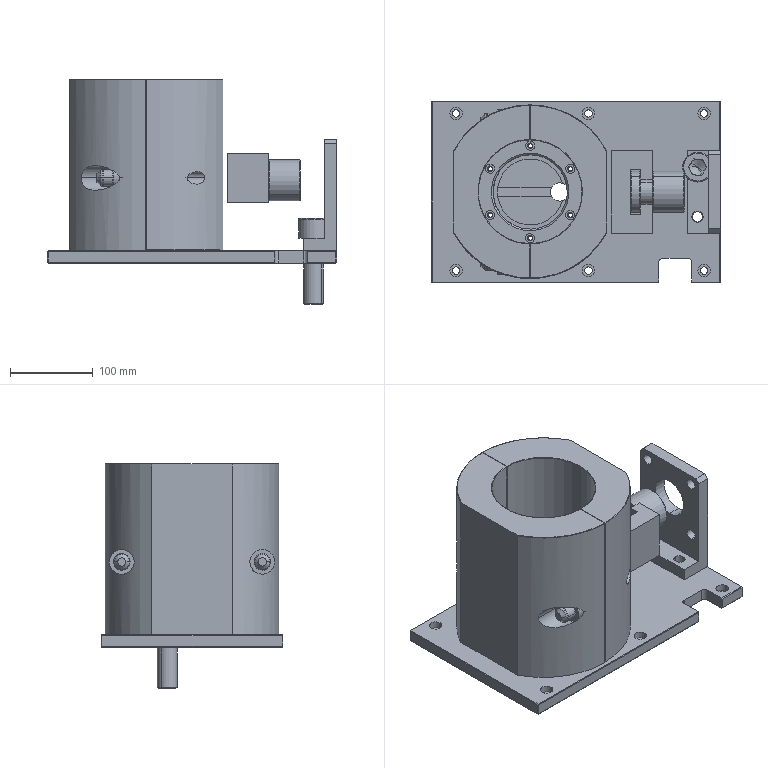Assembly | SolidWorks | mm | 12 component files | 13 solids | 524 faces | box 350 x 220 x 272 mm | volume 5983878 mm3 | cylinder 289 | plane 162 | cone 65 | torus 8 | commonest cylinder face diameters 15 x42 9 x42 20 x32 19.5 x20 6.8 x18 12 x16 5 x12 13.5 x12
Bill of materials:
GuideBushingLCHZ20-30 | 2 |  | Hollow cylindrical sleeve with a short, slightly larger-diameter collar at one end; plain through bore.
socket head cap screw_iso | 1 |  | Socket-head-style cap screw shape: cylindrical head with a hexagonal recess, and a plain cylindrical shank with a chamfered tip.
ZN-A-008 | 1 |  | Flat rectangular plate with many through holes of several sizes, a large central hole, a rectangular notch on one long edge, and a shallow circular groove plus a thin radial line on the top face.
ZN-A-009 | 1 |  | Axisymmetric spool-like part: a thin end flange and a longer main cylinder of the same outer diameter, joined by a reduced-diameter neck, with an axial hole.
ZN-A-010 | 1 |  | Thick split ring/collar block made of two halves split along a diametral plane, with a large central bore, two flat sides on the outer profile, and cross holes plus small holes on the outer faces.
ZN-A-012 | 1 |  | L-shaped bracket: a vertical rectangular plate with one large central hole and four smaller holes, plus a short horizontal base foot with two holes.
ZN-A-018 | 2 |  | Solid cylindrical pin/rod with a chamfered or tapered end and a small axial hole in the opposite flat end; faint circumferential lines along its length.
ZN-A-019 | 1 |  | Rectangular block with a T-shaped slot running through its full length, open on one face, and four through holes on the perpendicular faces.
ZN-A-020 | 1 |  | Flat flange ring with a large central bore, a small internal step/lip at the bore, and six evenly spaced through holes on a bolt circle.
ZN-A-027 | 1 |  | Thin flat annular ring with a large central opening, six evenly spaced through holes on a bolt circle, and small chamfers on the outer edges.
Mates:
1. coincident | ZN-A-008-1 face at (0, 0, 15) dir (0, 0, 1) | ZN-A-012-1 face at (633.392, 282.499, 15) dir (0, 0, -1)
2. width | ZN-A-008-1 face at (298.392, 122.499, 15) dir (0, -1, 0) | ZN-A-008-1 face at (298.392, 342.499, 15) dir (0, 1, 0) | ZN-A-012-1 face at (633.392, 282.499, 150) dir (0, 1, 0) | ZN-A-012-1 face at (633.392, 182.499, 150) dir (0, -1, 0)
3. concentric | ZN-A-009-1 face at (539.392, 232.499, 100) dir (1, 0, 0) r 25 | ZN-A-012-1 face at (608.392, 232.499, 100) dir (1, 0, 0) r 24
4. concentric | ZN-A-012-1 face at (620.392, 262.499, 30) dir (0, 0, 1) r 6.75 | socket head cap screw_iso-6 face at (620.392, 262.499, 85.75) dir (0, 0, 1) r 12
5. coincident | ZN-A-012-1 face at (633.392, 182.499, 30) dir (0, 0, 1) | socket head cap screw_iso-6 face at (610.547, 247.43, 30) dir (0, 0, -1)
6. concentric | ZN-A-008-1 face at (620.392, 202.499, 15) dir (0, 0, 1) r 6 | ZN-A-012-1 face at (620.392, 202.499, 30) dir (0, 0, 1) r 6.75
7. concentric | ZN-A-010-1 face at (510.892, 271.499, 84) dir (1, 0, 0) r 3.4 | ZN-A-019-1 face at (565.892, 271.499, 84) dir (1, 0, 0) r 7.5
8. concentric | ZN-A-010-1 face at (510.892, 193.499, 84) dir (1, 0, 0) r 3.4 | ZN-A-019-1 face at (565.892, 193.499, 84) dir (1, 0, 0) r 4.5
9. width | ZN-A-019-1 face at (565.892, 216.999, 133) dir (0, 1, 0) | ZN-A-019-1 face at (565.892, 247.999, 133) dir (0, -1, 0) | ZN-A-009-1 face at (539.392, 232.499, 100) dir (-1, 0, 0) r 15
10. concentric | ZN-A-010-1 face at (438.392, 317.499, 103) dir (-1, 0, 0) r 10 | ZN-A-018-1 face at (358.392, 317.499, 103) dir (1, 0, 0) r 10
11. coincident | ZN-A-010-1 face at (438.392, 317.499, 103) dir (-1, 0, 0) | ZN-A-018-1 face at (438.392, 317.499, 103) dir (1, 0, 0)
12. concentric | ZN-A-010-1 face at (438.392, 147.499, 103) dir (-1, 0, 0) r 10 | ZN-A-018-2 face at (358.392, 147.499, 103) dir (1, 0, 0) r 10
13. coincident | ZN-A-010-1 face at (438.392, 147.499, 103) dir (-1, 0, 0) | ZN-A-018-2 face at (438.392, 147.499, 103) dir (1, 0, 0)
14. coincident | ZN-A-008-1 face at (0, 0, 15) dir (0, 0, 1) | ZN-A-027-1 face at (417.892, 232.499, 15) dir (0, 0, -1)
15. concentric | ZN-A-010-1 face at (417.892, 232.499, 286.473) dir (0, 0, 1) r 62.775 | ZN-A-027-1 face at (417.892, 232.499, 15) dir (0, 0, 1) r 67
16. coincident | ZN-A-020-1 face at (417.892, 232.499, 30) dir (0, 0, -1) | ZN-A-027-1 face at (417.892, 232.499, 30) dir (0, 0, 1)
17. concentric | ZN-A-020-1 face at (369.328, 204.614, 52) dir (0, 0, 1) r 3.3 | ZN-A-027-1 face at (369.328, 204.614, 15) dir (0, 0, -1) r 7.5
18. concentric | ZN-A-020-1 face at (369.461, 260.614, 52) dir (0, 0, 1) r 3.3 | ZN-A-027-1 face at (369.461, 260.614, 15) dir (0, 0, -1) r 7.5
19. coincident | ZN-A-008-1 face at (0, 0, 15) dir (0, 0, 1) | ZN-A-010-1 face at (417.892, 337.499, 15) dir (0, 0, -1)
20. coincident | ZN-A-009-1 face at (565.892, 242.511, 88.83) dir (-1, 0, 0) | ZN-A-019-1 face at (565.892, 282.499, 133) dir (1, 0, 0)